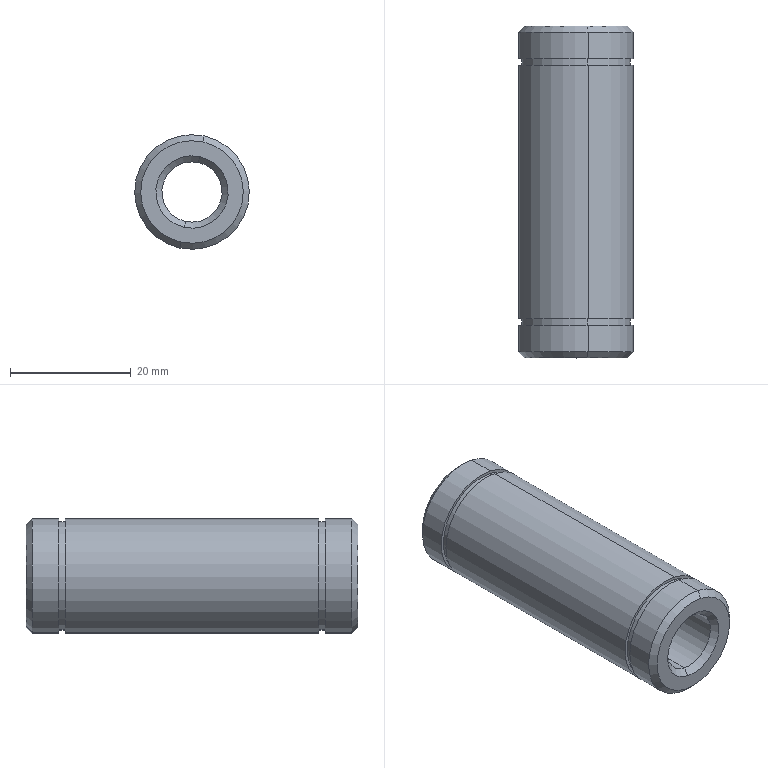Component | SolidWorks | LML10UU-2 | 1 solid | 26 faces | box 19 x 55 x 19 mm | volume 11119 mm3 | cylinder 12 | cone 8 | plane 6 | commonest cylinder face diameters 19 x6 18 x4 10 x2
build123d program:
from build123d import *

# Parameters (mm, degrees)
SKETCH1_R           = 9.5
BOSS_EXTRUDE1_DEPTH = 27.5
CUT_EXTRUDE1_REACH  = 58.617
SKETCH2_R           = 5
SKETCH3_W           = 0.5
SKETCH3_H           = 1.1
CHAMFER1_SIZE       = 1


with BuildPart() as part:
    # Sketch1 → Boss-Extrude1 (new, symmetric)
    with BuildSketch(Plane(origin=(0, 0, 0), x_dir=(1, 0, 0), z_dir=(0, 1, 0))):
        with Locations(Location((0, 0, 0), (0, 0, 270))):
            Circle(SKETCH1_R)
    extrude(amount=BOSS_EXTRUDE1_DEPTH, both=True)

    # Sketch2 → Cut-Extrude1 (cut, up to next)
    with BuildSketch(Plane(origin=(0, 27.5, 0), x_dir=(1, 0, 0), z_dir=(0, 1, 0)), mode=Mode.PRIVATE) as cut_extrude1_sk1:
        with Locations(Location((0, 0, 0), (0, 0, 270))):
            Circle(SKETCH2_R)
    cut_extrude1_tool1 = extrude(cut_extrude1_sk1.sketch, amount=-CUT_EXTRUDE1_REACH, mode=Mode.PRIVATE) & part.part
    add(cut_extrude1_tool1.solids().sort_by_distance((0, 27.5, 0))[0], mode=Mode.SUBTRACT)

    # Sketch3 → Cut-Revolve1 (revolve, cut)
    with BuildSketch(Plane.XY, mode=Mode.PRIVATE) as cut_revolve1_sk:
        with Locations((9.25, 21.55)):
            Rectangle(SKETCH3_W, SKETCH3_H)
        with Locations((9.25, -21.55)):
            Rectangle(SKETCH3_W, SKETCH3_H)
    revolve(cut_revolve1_sk.sketch.rotate(Axis((0, 27.5, 0), (0, -1, 0)), 90), axis=Axis((0, 27.5, 0), (0, -1, 0)), mode=Mode.SUBTRACT)

    # Chamfer1
    chamfer1_edges = [part.edges().sort_by_distance(p)[0] for p in [
        (0, -27.5, -9.5),
        (0, 27.5, -9.5),
        (0, 27.5, -5),
        (0, -27.5, -5),
    ]]
    chamfer(chamfer1_edges, length=CHAMFER1_SIZE)


solid = part.part

# Placed as in the assembly
solid = solid.moved(Location((-59.904, 281.499, -12), (0, 0, 0)))
STEP:
#1=COLOUR_RGB('',0.7922,0.8196,0.9333);
#2=FILL_AREA_STYLE_COLOUR('',#1);
#3=FILL_AREA_STYLE('',(#2));
#4=SURFACE_STYLE_FILL_AREA(#3);
#5=SURFACE_SIDE_STYLE('',(#4));
#6=SURFACE_STYLE_USAGE(.BOTH.,#5);
#7=PRESENTATION_STYLE_ASSIGNMENT((#6));
#8=CARTESIAN_POINT('',(-2.4,12.126,-0.6649));
#9=VERTEX_POINT('',#8);
#10=CARTESIAN_POINT('',(-2.317,12.126,-0.28));
#11=VERTEX_POINT('',#10);
#12=CARTESIAN_POINT('',(-2.358,12.126,-0.4724));
#13=DIRECTION('',(0.,1.,0.));
#14=DIRECTION('',(0.2108,0.,0.9775));
#15=AXIS2_PLACEMENT_3D('',#12,#13,#14);
#16=CIRCLE('',#15,0.1969);
#17=EDGE_CURVE('',#9,#11,#16,.T.);
#18=ORIENTED_EDGE('',*,*,#17,.F.);
#19=CARTESIAN_POINT('',(-2.408,12.165,-0.7034));
#20=VERTEX_POINT('',#19);
#21=CARTESIAN_POINT('',(-2.4,12.126,-0.6649));
#22=DIRECTION('',(-0.149,0.7071,-0.6912));
#23=VECTOR('',#22,39.37);
#24=LINE('',#21,#23);
#25=EDGE_CURVE('',#9,#20,#24,.T.);
#26=ORIENTED_EDGE('',*,*,#25,.T.);
#27=CARTESIAN_POINT('',(-2.309,12.165,-0.2415));
#28=VERTEX_POINT('',#27);
#29=CARTESIAN_POINT('',(-2.358,12.165,-0.4724));
#30=DIRECTION('',(0.,-1.,0.));
#31=DIRECTION('',(0.2108,0.,0.9775));
#32=AXIS2_PLACEMENT_3D('',#29,#30,#31);
#33=CIRCLE('',#32,0.2362);
#34=EDGE_CURVE('',#28,#20,#33,.T.);
#35=ORIENTED_EDGE('',*,*,#34,.F.);
#36=CARTESIAN_POINT('',(-2.317,12.126,-0.28));
#37=DIRECTION('',(0.149,0.7071,0.6912));
#38=VECTOR('',#37,39.37);
#39=LINE('',#36,#38);
#40=EDGE_CURVE('',#11,#28,#39,.T.);
#41=ORIENTED_EDGE('',*,*,#40,.F.);
#42=EDGE_LOOP('',(#18,#26,#35,#41));
#43=FACE_OUTER_BOUND('',#42,.T.);
#44=CARTESIAN_POINT('',(-2.358,12.126,-0.4724));
#45=DIRECTION('',(0.,1.,0.));
#46=DIRECTION('',(0.2108,0.,0.9775));
#47=AXIS2_PLACEMENT_3D('',#44,#45,#46);
#48=CONICAL_SURFACE('',#47,0.1969,0.7854);
#49=ADVANCED_FACE('',(#43),#48,.F.);
#50=CARTESIAN_POINT('',(-2.288,12.165,-0.1453));
#51=VERTEX_POINT('',#50);
#52=CARTESIAN_POINT('',(-2.429,12.165,-0.7996));
#53=VERTEX_POINT('',#52);
#54=CARTESIAN_POINT('',(-2.358,12.165,-0.4724));
#55=DIRECTION('',(0.,1.,0.));
#56=DIRECTION('',(0.2108,0.,0.9775));
#57=AXIS2_PLACEMENT_3D('',#54,#55,#56);
#58=CIRCLE('',#57,0.3346);
#59=EDGE_CURVE('',#51,#53,#58,.T.);
#60=ORIENTED_EDGE('',*,*,#59,.F.);
#61=CARTESIAN_POINT('',(-2.28,12.126,-0.1068));
#62=VERTEX_POINT('',#61);
#63=CARTESIAN_POINT('',(-2.288,12.165,-0.1453));
#64=DIRECTION('',(0.149,-0.7071,0.6912));
#65=VECTOR('',#64,39.37);
#66=LINE('',#63,#65);
#67=EDGE_CURVE('',#51,#62,#66,.T.);
#68=ORIENTED_EDGE('',*,*,#67,.T.);
#69=CARTESIAN_POINT('',(-2.437,12.126,-0.8381));
#70=VERTEX_POINT('',#69);
#71=CARTESIAN_POINT('',(-2.358,12.126,-0.4724));
#72=DIRECTION('',(0.,-1.,0.));
#73=DIRECTION('',(0.2108,0.,0.9775));
#74=AXIS2_PLACEMENT_3D('',#71,#72,#73);
#75=CIRCLE('',#74,0.374);
#76=EDGE_CURVE('',#70,#62,#75,.T.);
#77=ORIENTED_EDGE('',*,*,#76,.F.);
#78=CARTESIAN_POINT('',(-2.429,12.165,-0.7996));
#79=DIRECTION('',(-0.149,-0.7071,-0.6912));
#80=VECTOR('',#79,39.37);
#81=LINE('',#78,#80);
#82=EDGE_CURVE('',#53,#70,#81,.T.);
#83=ORIENTED_EDGE('',*,*,#82,.F.);
#84=EDGE_LOOP('',(#60,#68,#77,#83));
#85=FACE_OUTER_BOUND('',#84,.T.);
#86=CARTESIAN_POINT('',(-2.358,12.165,-0.4724));
#87=DIRECTION('',(0.,-1.,0.));
#88=DIRECTION('',(-0.2108,0.,-0.9775));
#89=AXIS2_PLACEMENT_3D('',#86,#87,#88);
#90=CONICAL_SURFACE('',#89,0.3346,0.7854);
#91=ADVANCED_FACE('',(#85),#90,.T.);
#92=CARTESIAN_POINT('',(-2.317,10.039,-0.28));
#93=VERTEX_POINT('',#92);
#94=CARTESIAN_POINT('',(-2.4,10.039,-0.6649));
#95=VERTEX_POINT('',#94);
#96=CARTESIAN_POINT('',(-2.358,10.039,-0.4724));
#97=DIRECTION('',(0.,-1.,0.));
#98=DIRECTION('',(0.2108,0.,0.9775));
#99=AXIS2_PLACEMENT_3D('',#96,#97,#98);
#100=CIRCLE('',#99,0.1969);
#101=EDGE_CURVE('',#93,#95,#100,.T.);
#102=ORIENTED_EDGE('',*,*,#101,.F.);
#103=CARTESIAN_POINT('',(-2.309,10.,-0.2415));
#104=VERTEX_POINT('',#103);
#105=CARTESIAN_POINT('',(-2.317,10.039,-0.28));
#106=DIRECTION('',(0.149,-0.7071,0.6912));
#107=VECTOR('',#106,39.37);
#108=LINE('',#105,#107);
#109=EDGE_CURVE('',#93,#104,#108,.T.);
#110=ORIENTED_EDGE('',*,*,#109,.T.);
#111=CARTESIAN_POINT('',(-2.408,10.,-0.7034));
#112=VERTEX_POINT('',#111);
#113=CARTESIAN_POINT('',(-2.358,10.,-0.4724));
#114=DIRECTION('',(0.,1.,0.));
#115=DIRECTION('',(0.2108,0.,0.9775));
#116=AXIS2_PLACEMENT_3D('',#113,#114,#115);
#117=CIRCLE('',#116,0.2362);
#118=EDGE_CURVE('',#112,#104,#117,.T.);
#119=ORIENTED_EDGE('',*,*,#118,.F.);
#120=CARTESIAN_POINT('',(-2.4,10.039,-0.6649));
#121=DIRECTION('',(-0.149,-0.7071,-0.6912));
#122=VECTOR('',#121,39.37);
#123=LINE('',#120,#122);
#124=EDGE_CURVE('',#95,#112,#123,.T.);
#125=ORIENTED_EDGE('',*,*,#124,.F.);
#126=EDGE_LOOP('',(#102,#110,#119,#125));
#127=FACE_OUTER_BOUND('',#126,.T.);
#128=CARTESIAN_POINT('',(-2.358,10.039,-0.4724));
#129=DIRECTION('',(0.,-1.,0.));
#130=DIRECTION('',(-0.2108,0.,-0.9775));
#131=AXIS2_PLACEMENT_3D('',#128,#129,#130);
#132=CONICAL_SURFACE('',#131,0.1969,0.7854);
#133=ADVANCED_FACE('',(#127),#132,.F.);
#134=CARTESIAN_POINT('',(-2.429,10.,-0.7996));
#135=VERTEX_POINT('',#134);
#136=CARTESIAN_POINT('',(-2.288,10.,-0.1453));
#137=VERTEX_POINT('',#136);
#138=CARTESIAN_POINT('',(-2.358,10.,-0.4724));
#139=DIRECTION('',(0.,-1.,0.));
#140=DIRECTION('',(0.2108,0.,0.9775));
#141=AXIS2_PLACEMENT_3D('',#138,#139,#140);
#142=CIRCLE('',#141,0.3346);
#143=EDGE_CURVE('',#135,#137,#142,.T.);
#144=ORIENTED_EDGE('',*,*,#143,.F.);
#145=CARTESIAN_POINT('',(-2.437,10.039,-0.8381));
#146=VERTEX_POINT('',#145);
#147=CARTESIAN_POINT('',(-2.437,10.039,-0.8381));
#148=DIRECTION('',(-0.149,0.7071,-0.6912));
#149=VECTOR('',#148,39.37);
#150=LINE('',#147,#149);
#151=EDGE_CURVE('',#135,#146,#150,.T.);
#152=ORIENTED_EDGE('',*,*,#151,.T.);
#153=CARTESIAN_POINT('',(-2.28,10.039,-0.1068));
#154=VERTEX_POINT('',#153);
#155=CARTESIAN_POINT('',(-2.358,10.039,-0.4724));
#156=DIRECTION('',(0.,1.,0.));
#157=DIRECTION('',(0.2108,0.,0.9775));
#158=AXIS2_PLACEMENT_3D('',#155,#156,#157);
#159=CIRCLE('',#158,0.374);
#160=EDGE_CURVE('',#154,#146,#159,.T.);
#161=ORIENTED_EDGE('',*,*,#160,.F.);
#162=CARTESIAN_POINT('',(-2.28,10.039,-0.1068));
#163=DIRECTION('',(0.149,0.7071,0.6912));
#164=VECTOR('',#163,39.37);
#165=LINE('',#162,#164);
#166=EDGE_CURVE('',#137,#154,#165,.T.);
#167=ORIENTED_EDGE('',*,*,#166,.F.);
#168=EDGE_LOOP('',(#144,#152,#161,#167));
#169=FACE_OUTER_BOUND('',#168,.T.);
#170=CARTESIAN_POINT('',(-2.358,10.039,-0.4724));
#171=DIRECTION('',(0.,1.,0.));
#172=DIRECTION('',(0.2108,0.,0.9775));
#173=AXIS2_PLACEMENT_3D('',#170,#171,#172);
#174=CONICAL_SURFACE('',#173,0.374,0.7854);
#175=ADVANCED_FACE('',(#169),#174,.T.);
#176=CARTESIAN_POINT('',(-2.284,10.213,-0.1261));
#177=VERTEX_POINT('',#176);
#178=CARTESIAN_POINT('',(-2.433,10.213,-0.8188));
#179=VERTEX_POINT('',#178);
#180=CARTESIAN_POINT('',(-2.358,10.213,-0.4724));
#181=DIRECTION('',(0.,1.,0.));
#182=DIRECTION('',(0.2108,0.,0.9775));
#183=AXIS2_PLACEMENT_3D('',#180,#181,#182);
#184=CIRCLE('',#183,0.3543);
#185=EDGE_CURVE('',#177,#179,#184,.T.);
#186=ORIENTED_EDGE('',*,*,#185,.T.);
#187=CARTESIAN_POINT('',(-2.433,10.256,-0.8188));
#188=VERTEX_POINT('',#187);
#189=CARTESIAN_POINT('',(-2.433,12.165,-0.8188));
#190=DIRECTION('',(0.,1.,0.));
#191=VECTOR('',#190,39.37);
#192=LINE('',#189,#191);
#193=EDGE_CURVE('',#179,#188,#192,.T.);
#194=ORIENTED_EDGE('',*,*,#193,.T.);
#195=CARTESIAN_POINT('',(-2.284,10.256,-0.1261));
#196=VERTEX_POINT('',#195);
#197=CARTESIAN_POINT('',(-2.358,10.256,-0.4724));
#198=DIRECTION('',(0.,1.,0.));
#199=DIRECTION('',(0.2108,0.,0.9775));
#200=AXIS2_PLACEMENT_3D('',#197,#198,#199);
#201=CIRCLE('',#200,0.3543);
#202=EDGE_CURVE('',#196,#188,#201,.T.);
#203=ORIENTED_EDGE('',*,*,#202,.F.);
#204=CARTESIAN_POINT('',(-2.284,12.165,-0.1261));
#205=DIRECTION('',(0.,1.,0.));
#206=VECTOR('',#205,39.37);
#207=LINE('',#204,#206);
#208=EDGE_CURVE('',#177,#196,#207,.T.);
#209=ORIENTED_EDGE('',*,*,#208,.F.);
#210=EDGE_LOOP('',(#186,#194,#203,#209));
#211=FACE_OUTER_BOUND('',#210,.T.);
#212=CARTESIAN_POINT('',(-2.358,12.165,-0.4724));
#213=DIRECTION('',(0.,1.,0.));
#214=DIRECTION('',(0.2108,0.,0.9775));
#215=AXIS2_PLACEMENT_3D('',#212,#213,#214);
#216=CYLINDRICAL_SURFACE('',#215,0.3543);
#217=ADVANCED_FACE('',(#211),#216,.T.);
#218=CARTESIAN_POINT('',(-2.284,11.909,-0.1261));
#219=VERTEX_POINT('',#218);
#220=CARTESIAN_POINT('',(-2.433,11.909,-0.8188));
#221=VERTEX_POINT('',#220);
#222=CARTESIAN_POINT('',(-2.358,11.909,-0.4724));
#223=DIRECTION('',(0.,1.,0.));
#224=DIRECTION('',(0.2108,0.,0.9775));
#225=AXIS2_PLACEMENT_3D('',#222,#223,#224);
#226=CIRCLE('',#225,0.3543);
#227=EDGE_CURVE('',#219,#221,#226,.T.);
#228=ORIENTED_EDGE('',*,*,#227,.T.);
#229=CARTESIAN_POINT('',(-2.433,11.953,-0.8188));
#230=VERTEX_POINT('',#229);
#231=CARTESIAN_POINT('',(-2.433,12.165,-0.8188));
#232=DIRECTION('',(0.,1.,0.));
#233=VECTOR('',#232,39.37);
#234=LINE('',#231,#233);
#235=EDGE_CURVE('',#221,#230,#234,.T.);
#236=ORIENTED_EDGE('',*,*,#235,.T.);
#237=CARTESIAN_POINT('',(-2.284,11.953,-0.1261));
#238=VERTEX_POINT('',#237);
#239=CARTESIAN_POINT('',(-2.358,11.953,-0.4724));
#240=DIRECTION('',(0.,1.,0.));
#241=DIRECTION('',(0.2108,0.,0.9775));
#242=AXIS2_PLACEMENT_3D('',#239,#240,#241);
#243=CIRCLE('',#242,0.3543);
#244=EDGE_CURVE('',#238,#230,#243,.T.);
#245=ORIENTED_EDGE('',*,*,#244,.F.);
#246=CARTESIAN_POINT('',(-2.284,12.165,-0.1261));
#247=DIRECTION('',(0.,1.,0.));
#248=VECTOR('',#247,39.37);
#249=LINE('',#246,#248);
#250=EDGE_CURVE('',#219,#238,#249,.T.);
#251=ORIENTED_EDGE('',*,*,#250,.F.);
#252=EDGE_LOOP('',(#228,#236,#245,#251));
#253=FACE_OUTER_BOUND('',#252,.T.);
#254=CARTESIAN_POINT('',(-2.358,12.165,-0.4724));
#255=DIRECTION('',(0.,1.,0.));
#256=DIRECTION('',(0.2108,0.,0.9775));
#257=AXIS2_PLACEMENT_3D('',#254,#255,#256);
#258=CYLINDRICAL_SURFACE('',#257,0.3543);
#259=ADVANCED_FACE('',(#253),#258,.T.);
#260=ORIENTED_EDGE('',*,*,#101,.T.);
#261=CARTESIAN_POINT('',(-2.4,10.,-0.6649));
#262=DIRECTION('',(0.,1.,0.));
#263=VECTOR('',#262,39.37);
#264=LINE('',#261,#263);
#265=EDGE_CURVE('',#95,#9,#264,.T.);
#266=ORIENTED_EDGE('',*,*,#265,.T.);
#267=ORIENTED_EDGE('',*,*,#17,.T.);
#268=CARTESIAN_POINT('',(-2.317,10.,-0.28));
#269=DIRECTION('',(0.,1.,0.));
#270=VECTOR('',#269,39.37);
#271=LINE('',#268,#270);
#272=EDGE_CURVE('',#93,#11,#271,.T.);
#273=ORIENTED_EDGE('',*,*,#272,.F.);
#274=EDGE_LOOP('',(#260,#266,#267,#273));
#275=FACE_OUTER_BOUND('',#274,.T.);
#276=CARTESIAN_POINT('',(-2.358,10.,-0.4724));
#277=DIRECTION('',(0.,1.,0.));
#278=DIRECTION('',(0.2108,0.,0.9775));
#279=AXIS2_PLACEMENT_3D('',#276,#277,#278);
#280=CYLINDRICAL_SURFACE('',#279,0.1969);
#281=ADVANCED_FACE('',(#275),#280,.F.);
#282=ORIENTED_EDGE('',*,*,#76,.T.);
#283=CARTESIAN_POINT('',(-2.28,11.953,-0.1068));
#284=VERTEX_POINT('',#283);
#285=CARTESIAN_POINT('',(-2.28,12.165,-0.1068));
#286=DIRECTION('',(0.,-1.,0.));
#287=VECTOR('',#286,39.37);
#288=LINE('',#285,#287);
#289=EDGE_CURVE('',#62,#284,#288,.T.);
#290=ORIENTED_EDGE('',*,*,#289,.T.);
#291=CARTESIAN_POINT('',(-2.437,11.953,-0.8381));
#292=VERTEX_POINT('',#291);
#293=CARTESIAN_POINT('',(-2.358,11.953,-0.4724));
#294=DIRECTION('',(0.,1.,0.));
#295=DIRECTION('',(0.2108,0.,0.9775));
#296=AXIS2_PLACEMENT_3D('',#293,#294,#295);
#297=CIRCLE('',#296,0.374);
#298=EDGE_CURVE('',#284,#292,#297,.T.);
#299=ORIENTED_EDGE('',*,*,#298,.T.);
#300=CARTESIAN_POINT('',(-2.437,12.165,-0.8381));
#301=DIRECTION('',(0.,-1.,0.));
#302=VECTOR('',#301,39.37);
#303=LINE('',#300,#302);
#304=EDGE_CURVE('',#70,#292,#303,.T.);
#305=ORIENTED_EDGE('',*,*,#304,.F.);
#306=EDGE_LOOP('',(#282,#290,#299,#305));
#307=FACE_OUTER_BOUND('',#306,.T.);
#308=CARTESIAN_POINT('',(-2.358,12.165,-0.4724));
#309=DIRECTION('',(0.,-1.,0.));
#310=DIRECTION('',(-0.2108,0.,-0.9775));
#311=AXIS2_PLACEMENT_3D('',#308,#309,#310);
#312=CYLINDRICAL_SURFACE('',#311,0.374);
#313=ADVANCED_FACE('',(#307),#312,.T.);
#314=CARTESIAN_POINT('',(-2.28,11.909,-0.1068));
#315=VERTEX_POINT('',#314);
#316=CARTESIAN_POINT('',(-2.437,11.909,-0.8381));
#317=VERTEX_POINT('',#316);
#318=CARTESIAN_POINT('',(-2.358,11.909,-0.4724));
#319=DIRECTION('',(0.,1.,0.));
#320=DIRECTION('',(0.2108,0.,0.9775));
#321=AXIS2_PLACEMENT_3D('',#318,#319,#320);
#322=CIRCLE('',#321,0.374);
#323=EDGE_CURVE('',#315,#317,#322,.T.);
#324=ORIENTED_EDGE('',*,*,#323,.F.);
#325=CARTESIAN_POINT('',(-2.28,10.256,-0.1068));
#326=VERTEX_POINT('',#325);
#327=CARTESIAN_POINT('',(-2.28,12.165,-0.1068));
#328=DIRECTION('',(0.,-1.,0.));
#329=VECTOR('',#328,39.37);
#330=LINE('',#327,#329);
#331=EDGE_CURVE('',#315,#326,#330,.T.);
#332=ORIENTED_EDGE('',*,*,#331,.T.);
#333=CARTESIAN_POINT('',(-2.437,10.256,-0.8381));
#334=VERTEX_POINT('',#333);
#335=CARTESIAN_POINT('',(-2.358,10.256,-0.4724));
#336=DIRECTION('',(0.,1.,0.));
#337=DIRECTION('',(0.2108,0.,0.9775));
#338=AXIS2_PLACEMENT_3D('',#335,#336,#337);
#339=CIRCLE('',#338,0.374);
#340=EDGE_CURVE('',#326,#334,#339,.T.);
#341=ORIENTED_EDGE('',*,*,#340,.T.);
#342=CARTESIAN_POINT('',(-2.437,12.165,-0.8381));
#343=DIRECTION('',(0.,-1.,0.));
#344=VECTOR('',#343,39.37);
#345=LINE('',#342,#344);
#346=EDGE_CURVE('',#317,#334,#345,.T.);
#347=ORIENTED_EDGE('',*,*,#346,.F.);
#348=EDGE_LOOP('',(#324,#332,#341,#347));
#349=FACE_OUTER_BOUND('',#348,.T.);
#350=CARTESIAN_POINT('',(-2.358,12.165,-0.4724));
#351=DIRECTION('',(0.,-1.,0.));
#352=DIRECTION('',(-0.2108,0.,-0.9775));
#353=AXIS2_PLACEMENT_3D('',#350,#351,#352);
#354=CYLINDRICAL_SURFACE('',#353,0.374);
#355=ADVANCED_FACE('',(#349),#354,.T.);
#356=CARTESIAN_POINT('',(-2.28,10.213,-0.1068));
#357=VERTEX_POINT('',#356);
#358=CARTESIAN_POINT('',(-2.437,10.213,-0.8381));
#359=VERTEX_POINT('',#358);
#360=CARTESIAN_POINT('',(-2.358,10.213,-0.4724));
#361=DIRECTION('',(0.,1.,0.));
#362=DIRECTION('',(0.2108,0.,0.9775));
#363=AXIS2_PLACEMENT_3D('',#360,#361,#362);
#364=CIRCLE('',#363,0.374);
#365=EDGE_CURVE('',#357,#359,#364,.T.);
#366=ORIENTED_EDGE('',*,*,#365,.F.);
#367=CARTESIAN_POINT('',(-2.28,12.165,-0.1068));
#368=DIRECTION('',(0.,-1.,0.));
#369=VECTOR('',#368,39.37);
#370=LINE('',#367,#369);
#371=EDGE_CURVE('',#357,#154,#370,.T.);
#372=ORIENTED_EDGE('',*,*,#371,.T.);
#373=ORIENTED_EDGE('',*,*,#160,.T.);
#374=CARTESIAN_POINT('',(-2.437,12.165,-0.8381));
#375=DIRECTION('',(0.,-1.,0.));
#376=VECTOR('',#375,39.37);
#377=LINE('',#374,#376);
#378=EDGE_CURVE('',#359,#146,#377,.T.);
#379=ORIENTED_EDGE('',*,*,#378,.F.);
#380=EDGE_LOOP('',(#366,#372,#373,#379));
#381=FACE_OUTER_BOUND('',#380,.T.);
#382=CARTESIAN_POINT('',(-2.358,12.165,-0.4724));
#383=DIRECTION('',(0.,-1.,0.));
#384=DIRECTION('',(-0.2108,0.,-0.9775));
#385=AXIS2_PLACEMENT_3D('',#382,#383,#384);
#386=CYLINDRICAL_SURFACE('',#385,0.374);
#387=ADVANCED_FACE('',(#381),#386,.T.);
#388=ORIENTED_EDGE('',*,*,#371,.F.);
#389=CARTESIAN_POINT('',(-2.358,10.213,-0.4724));
#390=DIRECTION('',(0.,1.,0.));
#391=DIRECTION('',(0.2108,0.,0.9775));
#392=AXIS2_PLACEMENT_3D('',#389,#390,#391);
#393=CIRCLE('',#392,0.374);
#394=EDGE_CURVE('',#359,#357,#393,.T.);
#395=ORIENTED_EDGE('',*,*,#394,.F.);
#396=ORIENTED_EDGE('',*,*,#378,.T.);
#397=CARTESIAN_POINT('',(-2.358,10.039,-0.4724));
#398=DIRECTION('',(0.,1.,0.));
#399=DIRECTION('',(0.2108,0.,0.9775));
#400=AXIS2_PLACEMENT_3D('',#397,#398,#399);
#401=CIRCLE('',#400,0.374);
#402=EDGE_CURVE('',#146,#154,#401,.T.);
#403=ORIENTED_EDGE('',*,*,#402,.T.);
#404=EDGE_LOOP('',(#388,#395,#396,#403));
#405=FACE_OUTER_BOUND('',#404,.T.);
#406=CARTESIAN_POINT('',(-2.358,12.165,-0.4724));
#407=DIRECTION('',(0.,-1.,0.));
#408=DIRECTION('',(-0.2108,0.,-0.9775));
#409=AXIS2_PLACEMENT_3D('',#406,#407,#408);
#410=CYLINDRICAL_SURFACE('',#409,0.374);
#411=ADVANCED_FACE('',(#405),#410,.T.);
#412=ORIENTED_EDGE('',*,*,#331,.F.);
#413=CARTESIAN_POINT('',(-2.358,11.909,-0.4724));
#414=DIRECTION('',(0.,1.,0.));
#415=DIRECTION('',(0.2108,0.,0.9775));
#416=AXIS2_PLACEMENT_3D('',#413,#414,#415);
#417=CIRCLE('',#416,0.374);
#418=EDGE_CURVE('',#317,#315,#417,.T.);
#419=ORIENTED_EDGE('',*,*,#418,.F.);
#420=ORIENTED_EDGE('',*,*,#346,.T.);
#421=CARTESIAN_POINT('',(-2.358,10.256,-0.4724));
#422=DIRECTION('',(0.,1.,0.));
#423=DIRECTION('',(0.2108,0.,0.9775));
#424=AXIS2_PLACEMENT_3D('',#421,#422,#423);
#425=CIRCLE('',#424,0.374);
#426=EDGE_CURVE('',#334,#326,#425,.T.);
#427=ORIENTED_EDGE('',*,*,#426,.T.);
#428=EDGE_LOOP('',(#412,#419,#420,#427));
#429=FACE_OUTER_BOUND('',#428,.T.);
#430=CARTESIAN_POINT('',(-2.358,12.165,-0.4724));
#431=DIRECTION('',(0.,-1.,0.));
#432=DIRECTION('',(-0.2108,0.,-0.9775));
#433=AXIS2_PLACEMENT_3D('',#430,#431,#432);
#434=CYLINDRICAL_SURFACE('',#433,0.374);
#435=ADVANCED_FACE('',(#429),#434,.T.);
#436=ORIENTED_EDGE('',*,*,#289,.F.);
#437=CARTESIAN_POINT('',(-2.358,12.126,-0.4724));
#438=DIRECTION('',(0.,-1.,0.));
#439=DIRECTION('',(0.2108,0.,0.9775));
#440=AXIS2_PLACEMENT_3D('',#437,#438,#439);
#441=CIRCLE('',#440,0.374);
#442=EDGE_CURVE('',#62,#70,#441,.T.);
#443=ORIENTED_EDGE('',*,*,#442,.T.);
#444=ORIENTED_EDGE('',*,*,#304,.T.);
#445=CARTESIAN_POINT('',(-2.358,11.953,-0.4724));
#446=DIRECTION('',(0.,1.,0.));
#447=DIRECTION('',(0.2108,0.,0.9775));
#448=AXIS2_PLACEMENT_3D('',#445,#446,#447);
#449=CIRCLE('',#448,0.374);
#450=EDGE_CURVE('',#292,#284,#449,.T.);
#451=ORIENTED_EDGE('',*,*,#450,.T.);
#452=EDGE_LOOP('',(#436,#443,#444,#451));
#453=FACE_OUTER_BOUND('',#452,.T.);
#454=CARTESIAN_POINT('',(-2.358,12.165,-0.4724));
#455=DIRECTION('',(0.,-1.,0.));
#456=DIRECTION('',(-0.2108,0.,-0.9775));
#457=AXIS2_PLACEMENT_3D('',#454,#455,#456);
#458=CYLINDRICAL_SURFACE('',#457,0.374);
#459=ADVANCED_FACE('',(#453),#458,.T.);
#460=CARTESIAN_POINT('',(-2.358,12.165,-0.4724));
#461=DIRECTION('',(0.,1.,0.));
#462=DIRECTION('',(0.2108,0.,0.9775));
#463=AXIS2_PLACEMENT_3D('',#460,#461,#462);
#464=CIRCLE('',#463,0.3346);
#465=EDGE_CURVE('',#53,#51,#464,.T.);
#466=ORIENTED_EDGE('',*,*,#465,.T.);
#467=ORIENTED_EDGE('',*,*,#59,.T.);
#468=EDGE_LOOP('',(#466,#467));
#469=FACE_OUTER_BOUND('',#468,.T.);
#470=ORIENTED_EDGE('',*,*,#34,.T.);
#471=CARTESIAN_POINT('',(-2.358,12.165,-0.4724));
#472=DIRECTION('',(0.,-1.,0.));
#473=DIRECTION('',(0.2108,0.,0.9775));
#474=AXIS2_PLACEMENT_3D('',#471,#472,#473);
#475=CIRCLE('',#474,0.2362);
#476=EDGE_CURVE('',#20,#28,#475,.T.);
#477=ORIENTED_EDGE('',*,*,#476,.T.);
#478=EDGE_LOOP('',(#470,#477));
#479=FACE_BOUND('',#478,.T.);
#480=CARTESIAN_POINT('',(-2.358,12.165,-0.4724));
#481=DIRECTION('',(0.,1.,0.));
#482=DIRECTION('',(0.2108,0.,0.9775));
#483=AXIS2_PLACEMENT_3D('',#480,#481,#482);
#484=PLANE('',#483);
#485=ADVANCED_FACE('',(#469,#479),#484,.T.);
#486=CARTESIAN_POINT('',(-2.358,10.,-0.4724));
#487=DIRECTION('',(0.,-1.,0.));
#488=DIRECTION('',(0.2108,0.,0.9775));
#489=AXIS2_PLACEMENT_3D('',#486,#487,#488);
#490=CIRCLE('',#489,0.3346);
#491=EDGE_CURVE('',#137,#135,#490,.T.);
#492=ORIENTED_EDGE('',*,*,#491,.T.);
#493=ORIENTED_EDGE('',*,*,#143,.T.);
#494=EDGE_LOOP('',(#492,#493));
#495=FACE_OUTER_BOUND('',#494,.T.);
#496=ORIENTED_EDGE('',*,*,#118,.T.);
#497=CARTESIAN_POINT('',(-2.358,10.,-0.4724));
#498=DIRECTION('',(0.,1.,0.));
#499=DIRECTION('',(0.2108,0.,0.9775));
#500=AXIS2_PLACEMENT_3D('',#497,#498,#499);
#501=CIRCLE('',#500,0.2362);
#502=EDGE_CURVE('',#104,#112,#501,.T.);
#503=ORIENTED_EDGE('',*,*,#502,.T.);
#504=EDGE_LOOP('',(#496,#503));
#505=FACE_BOUND('',#504,.T.);
#506=CARTESIAN_POINT('',(-2.358,10.,-0.4724));
#507=DIRECTION('',(0.,1.,0.));
#508=DIRECTION('',(0.2108,0.,0.9775));
#509=AXIS2_PLACEMENT_3D('',#506,#507,#508);
#510=PLANE('',#509);
#511=ADVANCED_FACE('',(#495,#505),#510,.F.);
#512=ORIENTED_EDGE('',*,*,#265,.F.);
#513=CARTESIAN_POINT('',(-2.358,10.039,-0.4724));
#514=DIRECTION('',(0.,-1.,0.));
#515=DIRECTION('',(0.2108,0.,0.9775));
#516=AXIS2_PLACEMENT_3D('',#513,#514,#515);
#517=CIRCLE('',#516,0.1969);
#518=EDGE_CURVE('',#95,#93,#517,.T.);
#519=ORIENTED_EDGE('',*,*,#518,.T.);
#520=ORIENTED_EDGE('',*,*,#272,.T.);
#521=CARTESIAN_POINT('',(-2.358,12.126,-0.4724));
#522=DIRECTION('',(0.,1.,0.));
#523=DIRECTION('',(0.2108,0.,0.9775));
#524=AXIS2_PLACEMENT_3D('',#521,#522,#523);
#525=CIRCLE('',#524,0.1969);
#526=EDGE_CURVE('',#11,#9,#525,.T.);
#527=ORIENTED_EDGE('',*,*,#526,.T.);
#528=EDGE_LOOP('',(#512,#519,#520,#527));
#529=FACE_OUTER_BOUND('',#528,.T.);
#530=CARTESIAN_POINT('',(-2.358,10.,-0.4724));
#531=DIRECTION('',(0.,1.,0.));
#532=DIRECTION('',(0.2108,0.,0.9775));
#533=AXIS2_PLACEMENT_3D('',#530,#531,#532);
#534=CYLINDRICAL_SURFACE('',#533,0.1969);
#535=ADVANCED_FACE('',(#529),#534,.F.);
#536=ORIENTED_EDGE('',*,*,#418,.T.);
#537=ORIENTED_EDGE('',*,*,#323,.T.);
#538=EDGE_LOOP('',(#536,#537));
#539=FACE_OUTER_BOUND('',#538,.T.);
#540=ORIENTED_EDGE('',*,*,#227,.F.);
#541=CARTESIAN_POINT('',(-2.358,11.909,-0.4724));
#542=DIRECTION('',(0.,1.,0.));
#543=DIRECTION('',(0.2108,0.,0.9775));
#544=AXIS2_PLACEMENT_3D('',#541,#542,#543);
#545=CIRCLE('',#544,0.3543);
#546=EDGE_CURVE('',#221,#219,#545,.T.);
#547=ORIENTED_EDGE('',*,*,#546,.F.);
#548=EDGE_LOOP('',(#540,#547));
#549=FACE_BOUND('',#548,.T.);
#550=CARTESIAN_POINT('',(-1.993,11.909,-0.5513));
#551=DIRECTION('',(0.,1.,0.));
#552=DIRECTION('',(0.2108,0.,0.9775));
#553=AXIS2_PLACEMENT_3D('',#550,#551,#552);
#554=PLANE('',#553);
#555=ADVANCED_FACE('',(#539,#549),#554,.T.);
#556=ORIENTED_EDGE('',*,*,#235,.F.);
#557=ORIENTED_EDGE('',*,*,#546,.T.);
#558=ORIENTED_EDGE('',*,*,#250,.T.);
#559=CARTESIAN_POINT('',(-2.358,11.953,-0.4724));
#560=DIRECTION('',(0.,1.,0.));
#561=DIRECTION('',(0.2108,0.,0.9775));
#562=AXIS2_PLACEMENT_3D('',#559,#560,#561);
#563=CIRCLE('',#562,0.3543);
#564=EDGE_CURVE('',#230,#238,#563,.T.);
#565=ORIENTED_EDGE('',*,*,#564,.F.);
#566=EDGE_LOOP('',(#556,#557,#558,#565));
#567=FACE_OUTER_BOUND('',#566,.T.);
#568=CARTESIAN_POINT('',(-2.358,12.165,-0.4724));
#569=DIRECTION('',(0.,1.,0.));
#570=DIRECTION('',(0.2108,0.,0.9775));
#571=AXIS2_PLACEMENT_3D('',#568,#569,#570);
#572=CYLINDRICAL_SURFACE('',#571,0.3543);
#573=ADVANCED_FACE('',(#567),#572,.T.);
#574=ORIENTED_EDGE('',*,*,#244,.T.);
#575=ORIENTED_EDGE('',*,*,#564,.T.);
#576=EDGE_LOOP('',(#574,#575));
#577=FACE_BOUND('',#576,.T.);
#578=ORIENTED_EDGE('',*,*,#450,.F.);
#579=ORIENTED_EDGE('',*,*,#298,.F.);
#580=EDGE_LOOP('',(#578,#579));
#581=FACE_OUTER_BOUND('',#580,.T.);
#582=CARTESIAN_POINT('',(-1.993,11.953,-0.5513));
#583=DIRECTION('',(0.,-1.,0.));
#584=DIRECTION('',(-0.2108,0.,-0.9775));
#585=AXIS2_PLACEMENT_3D('',#582,#583,#584);
#586=PLANE('',#585);
#587=ADVANCED_FACE('',(#577,#581),#586,.T.);
#588=ORIENTED_EDGE('',*,*,#394,.T.);
#589=ORIENTED_EDGE('',*,*,#365,.T.);
#590=EDGE_LOOP('',(#588,#589));
#591=FACE_OUTER_BOUND('',#590,.T.);
#592=ORIENTED_EDGE('',*,*,#185,.F.);
#593=CARTESIAN_POINT('',(-2.358,10.213,-0.4724));
#594=DIRECTION('',(0.,1.,0.));
#595=DIRECTION('',(0.2108,0.,0.9775));
#596=AXIS2_PLACEMENT_3D('',#593,#594,#595);
#597=CIRCLE('',#596,0.3543);
#598=EDGE_CURVE('',#179,#177,#597,.T.);
#599=ORIENTED_EDGE('',*,*,#598,.F.);
#600=EDGE_LOOP('',(#592,#599));
#601=FACE_BOUND('',#600,.T.);
#602=CARTESIAN_POINT('',(-1.993,10.213,-0.5513));
#603=DIRECTION('',(0.,1.,0.));
#604=DIRECTION('',(0.2108,0.,0.9775));
#605=AXIS2_PLACEMENT_3D('',#602,#603,#604);
#606=PLANE('',#605);
#607=ADVANCED_FACE('',(#591,#601),#606,.T.);
#608=ORIENTED_EDGE('',*,*,#193,.F.);
#609=ORIENTED_EDGE('',*,*,#598,.T.);
#610=ORIENTED_EDGE('',*,*,#208,.T.);
#611=CARTESIAN_POINT('',(-2.358,10.256,-0.4724));
#612=DIRECTION('',(0.,1.,0.));
#613=DIRECTION('',(0.2108,0.,0.9775));
#614=AXIS2_PLACEMENT_3D('',#611,#612,#613);
#615=CIRCLE('',#614,0.3543);
#616=EDGE_CURVE('',#188,#196,#615,.T.);
#617=ORIENTED_EDGE('',*,*,#616,.F.);
#618=EDGE_LOOP('',(#608,#609,#610,#617));
#619=FACE_OUTER_BOUND('',#618,.T.);
#620=CARTESIAN_POINT('',(-2.358,12.165,-0.4724));
#621=DIRECTION('',(0.,1.,0.));
#622=DIRECTION('',(0.2108,0.,0.9775));
#623=AXIS2_PLACEMENT_3D('',#620,#621,#622);
#624=CYLINDRICAL_SURFACE('',#623,0.3543);
#625=ADVANCED_FACE('',(#619),#624,.T.);
#626=ORIENTED_EDGE('',*,*,#202,.T.);
#627=ORIENTED_EDGE('',*,*,#616,.T.);
#628=EDGE_LOOP('',(#626,#627));
#629=FACE_BOUND('',#628,.T.);
#630=ORIENTED_EDGE('',*,*,#426,.F.);
#631=ORIENTED_EDGE('',*,*,#340,.F.);
#632=EDGE_LOOP('',(#630,#631));
#633=FACE_OUTER_BOUND('',#632,.T.);
#634=CARTESIAN_POINT('',(-1.993,10.256,-0.5513));
#635=DIRECTION('',(0.,-1.,0.));
#636=DIRECTION('',(-0.2108,0.,-0.9775));
#637=AXIS2_PLACEMENT_3D('',#634,#635,#636);
#638=PLANE('',#637);
#639=ADVANCED_FACE('',(#629,#633),#638,.T.);
#640=ORIENTED_EDGE('',*,*,#151,.F.);
#641=ORIENTED_EDGE('',*,*,#491,.F.);
#642=ORIENTED_EDGE('',*,*,#166,.T.);
#643=ORIENTED_EDGE('',*,*,#402,.F.);
#644=EDGE_LOOP('',(#640,#641,#642,#643));
#645=FACE_OUTER_BOUND('',#644,.T.);
#646=CARTESIAN_POINT('',(-2.358,10.039,-0.4724));
#647=DIRECTION('',(0.,1.,0.));
#648=DIRECTION('',(0.2108,0.,0.9775));
#649=AXIS2_PLACEMENT_3D('',#646,#647,#648);
#650=CONICAL_SURFACE('',#649,0.374,0.7854);
#651=ADVANCED_FACE('',(#645),#650,.T.);
#652=ORIENTED_EDGE('',*,*,#109,.F.);
#653=ORIENTED_EDGE('',*,*,#518,.F.);
#654=ORIENTED_EDGE('',*,*,#124,.T.);
#655=ORIENTED_EDGE('',*,*,#502,.F.);
#656=EDGE_LOOP('',(#652,#653,#654,#655));
#657=FACE_OUTER_BOUND('',#656,.T.);
#658=CARTESIAN_POINT('',(-2.358,10.039,-0.4724));
#659=DIRECTION('',(0.,-1.,0.));
#660=DIRECTION('',(-0.2108,0.,-0.9775));
#661=AXIS2_PLACEMENT_3D('',#658,#659,#660);
#662=CONICAL_SURFACE('',#661,0.1969,0.7854);
#663=ADVANCED_FACE('',(#657),#662,.F.);
#664=ORIENTED_EDGE('',*,*,#67,.F.);
#665=ORIENTED_EDGE('',*,*,#465,.F.);
#666=ORIENTED_EDGE('',*,*,#82,.T.);
#667=ORIENTED_EDGE('',*,*,#442,.F.);
#668=EDGE_LOOP('',(#664,#665,#666,#667));
#669=FACE_OUTER_BOUND('',#668,.T.);
#670=CARTESIAN_POINT('',(-2.358,12.165,-0.4724));
#671=DIRECTION('',(0.,-1.,0.));
#672=DIRECTION('',(-0.2108,0.,-0.9775));
#673=AXIS2_PLACEMENT_3D('',#670,#671,#672);
#674=CONICAL_SURFACE('',#673,0.3346,0.7854);
#675=ADVANCED_FACE('',(#669),#674,.T.);
#676=ORIENTED_EDGE('',*,*,#25,.F.);
#677=ORIENTED_EDGE('',*,*,#526,.F.);
#678=ORIENTED_EDGE('',*,*,#40,.T.);
#679=ORIENTED_EDGE('',*,*,#476,.F.);
#680=EDGE_LOOP('',(#676,#677,#678,#679));
#681=FACE_OUTER_BOUND('',#680,.T.);
#682=CARTESIAN_POINT('',(-2.358,12.126,-0.4724));
#683=DIRECTION('',(0.,1.,0.));
#684=DIRECTION('',(0.2108,0.,0.9775));
#685=AXIS2_PLACEMENT_3D('',#682,#683,#684);
#686=CONICAL_SURFACE('',#685,0.1969,0.7854);
#687=ADVANCED_FACE('',(#681),#686,.F.);
#688=CLOSED_SHELL('',(#49,#91,#133,#175,#217,#259,#281,#313,#355,#387,#411,#435,#459,#485,#511,#535,#555,#573,#587,#607,#625,#639,#651,#663,#675,#687));
#689=MANIFOLD_SOLID_BREP('',#688);
#690=STYLED_ITEM('',(#7),#689);
#691=PRESENTATION_LAYER_ASSIGNMENT('','',(#690));
#692=(LENGTH_UNIT()NAMED_UNIT(*)SI_UNIT($,.METRE.));
#693=LENGTH_MEASURE_WITH_UNIT(LENGTH_MEASURE(0.0254),#692);
#694=DIMENSIONAL_EXPONENTS(1.,0.,0.,0.,0.,0.,0.);
#695=(CONVERSION_BASED_UNIT('',#693)LENGTH_UNIT()NAMED_UNIT(#694));
#696=UNCERTAINTY_MEASURE_WITH_UNIT(LENGTH_MEASURE(0.00001),#695,'','');
#697=(NAMED_UNIT(*)PLANE_ANGLE_UNIT()SI_UNIT($,.RADIAN.));
#698=(NAMED_UNIT(*)SI_UNIT($,.STERADIAN.)SOLID_ANGLE_UNIT());
#699=(GEOMETRIC_REPRESENTATION_CONTEXT(3)GLOBAL_UNCERTAINTY_ASSIGNED_CONTEXT((#696))GLOBAL_UNIT_ASSIGNED_CONTEXT((#695,#697,#698))REPRESENTATION_CONTEXT('',''));
#700=MECHANICAL_DESIGN_GEOMETRIC_PRESENTATION_REPRESENTATION('',(#690),#699);
#701=CARTESIAN_POINT('',(0.,0.,0.));
#702=DIRECTION('',(0.,0.,1.));
#703=DIRECTION('',(1.,0.,0.));
#704=AXIS2_PLACEMENT_3D('',#701,#702,#703);
#705=(LENGTH_UNIT()NAMED_UNIT(*)SI_UNIT($,.METRE.));
#706=LENGTH_MEASURE_WITH_UNIT(LENGTH_MEASURE(0.0254),#705);
#707=DIMENSIONAL_EXPONENTS(1.,0.,0.,0.,0.,0.,0.);
#708=(CONVERSION_BASED_UNIT('',#706)LENGTH_UNIT()NAMED_UNIT(#707));
#709=UNCERTAINTY_MEASURE_WITH_UNIT(LENGTH_MEASURE(0.00001),#708,'','');
#710=(NAMED_UNIT(*)PLANE_ANGLE_UNIT()SI_UNIT($,.RADIAN.));
#711=(NAMED_UNIT(*)SI_UNIT($,.STERADIAN.)SOLID_ANGLE_UNIT());
#712=(GEOMETRIC_REPRESENTATION_CONTEXT(3)GLOBAL_UNCERTAINTY_ASSIGNED_CONTEXT((#709))GLOBAL_UNIT_ASSIGNED_CONTEXT((#708,#710,#711))REPRESENTATION_CONTEXT('',''));
#713=ADVANCED_BREP_SHAPE_REPRESENTATION('',(#689,#704),#712);